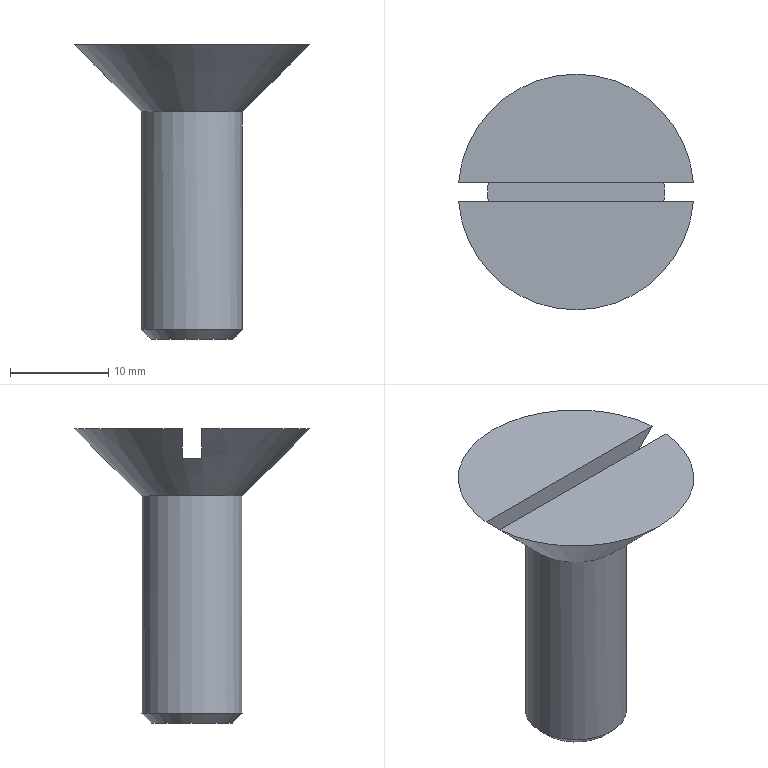Component | NX | COUNTER_SUNK_SCREW | 1 solid | 9 faces | box 23.92 x 24 x 30 mm | volume 3455 mm3 | plane 6 | cone 2 | cylinder 1 | commonest cylinder face diameters 10.3 x1
STEP:
#1=CARTESIAN_POINT('',(0.,0.,0.));
#2=DIRECTION('',(0.,0.,1.));
#3=DIRECTION('',(1.,0.,0.));
#4=AXIS2_PLACEMENT_3D('',#1,#2,#3);
#5=CARTESIAN_POINT('',(5.132,239.571,313.65));
#6=VERTEX_POINT('',#5);
#7=CARTESIAN_POINT('',(-5.15,240.,313.65));
#8=VERTEX_POINT('',#7);
#9=CARTESIAN_POINT('',(0.,240.,313.65));
#10=DIRECTION('',(0.,0.,-1.));
#11=DIRECTION('',(-1.,0.,0.));
#12=AXIS2_PLACEMENT_3D('',#9,#10,#11);
#13=CIRCLE('',#12,5.15);
#14=CARTESIAN_POINT('',(0.,240.,313.65));
#15=DIRECTION('',(0.,0.,1.));
#16=DIRECTION('',(1.,0.,0.));
#17=AXIS2_PLACEMENT_3D('',#14,#15,#16);
#18=CONICAL_SURFACE('',#17,5.15,0.7854);
#19=CARTESIAN_POINT('',(15.708,0.));
#20=DIRECTION('',(-1.,0.));
#21=VECTOR('',#20,1.);
#22=LINE('',#19,#21);
#23=(GEOMETRIC_REPRESENTATION_CONTEXT(2)PARAMETRIC_REPRESENTATION_CONTEXT()REPRESENTATION_CONTEXT('',''));
#24=DEFINITIONAL_REPRESENTATION('',(#22),#23);
#25=PCURVE('',#18,#24);
#26=CARTESIAN_POINT('',(0.,240.,290.5));
#27=DIRECTION('',(0.,0.,-1.));
#28=DIRECTION('',(-1.,0.,0.));
#29=AXIS2_PLACEMENT_3D('',#26,#27,#28);
#30=CYLINDRICAL_SURFACE('',#29,5.15);
#31=CARTESIAN_POINT('',(0.,-23.15));
#32=DIRECTION('',(1.,0.));
#33=VECTOR('',#32,1.);
#34=LINE('',#31,#33);
#35=(GEOMETRIC_REPRESENTATION_CONTEXT(2)PARAMETRIC_REPRESENTATION_CONTEXT()REPRESENTATION_CONTEXT('',''));
#36=DEFINITIONAL_REPRESENTATION('',(#34),#35);
#37=PCURVE('',#30,#36);
#38=SURFACE_CURVE('',#13,(#25,#37),.PCURVE_S1.);
#39=EDGE_CURVE('',#6,#8,#38,.T.);
#40=ORIENTED_EDGE('',*,*,#39,.F.);
#41=CARTESIAN_POINT('',(8.969,239.25,317.5));
#42=VERTEX_POINT('',#41);
#43=CARTESIAN_POINT('',(5.132,239.571,313.65));
#44=CARTESIAN_POINT('',(8.969,239.25,317.5));
#45=B_SPLINE_CURVE_WITH_KNOTS('',1,(#43,#44),.UNSPECIFIED.,.F.,.F.,(2,2),(0.,5.445),.PIECEWISE_BEZIER_KNOTS.);
#46=CARTESIAN_POINT('',(12.483,0.));
#47=DIRECTION('',(0.,1.));
#48=VECTOR('',#47,1.);
#49=LINE('',#46,#48);
#50=(GEOMETRIC_REPRESENTATION_CONTEXT(2)PARAMETRIC_REPRESENTATION_CONTEXT()REPRESENTATION_CONTEXT('',''));
#51=DEFINITIONAL_REPRESENTATION('',(#49),#50);
#52=PCURVE('',#18,#51);
#53=CARTESIAN_POINT('',(6.2,0.));
#54=DIRECTION('',(0.,1.));
#55=VECTOR('',#54,1.);
#56=LINE('',#53,#55);
#57=(GEOMETRIC_REPRESENTATION_CONTEXT(2)PARAMETRIC_REPRESENTATION_CONTEXT()REPRESENTATION_CONTEXT('',''));
#58=DEFINITIONAL_REPRESENTATION('',(#56),#57);
#59=PCURVE('',#18,#58);
#60=SEAM_CURVE('',#45,(#52,#59),.PCURVE_S1.);
#61=EDGE_CURVE('',#6,#42,#60,.T.);
#62=ORIENTED_EDGE('',*,*,#61,.T.);
#63=CARTESIAN_POINT('',(8.944,239.,317.5));
#64=VERTEX_POINT('',#63);
#65=CARTESIAN_POINT('',(0.,240.,317.5));
#66=DIRECTION('',(0.,0.,-1.));
#67=DIRECTION('',(1.,0.,0.));
#68=AXIS2_PLACEMENT_3D('',#65,#66,#67);
#69=CIRCLE('',#68,9.);
#70=CARTESIAN_POINT('',(12.566,3.85));
#71=DIRECTION('',(-1.,0.));
#72=VECTOR('',#71,1.);
#73=LINE('',#70,#72);
#74=(GEOMETRIC_REPRESENTATION_CONTEXT(2)PARAMETRIC_REPRESENTATION_CONTEXT()REPRESENTATION_CONTEXT('',''));
#75=DEFINITIONAL_REPRESENTATION('',(#73),#74);
#76=PCURVE('',#18,#75);
#77=CARTESIAN_POINT('',(213.,239.,317.5));
#78=DIRECTION('',(0.,0.,1.));
#79=DIRECTION('',(1.,0.,0.));
#80=AXIS2_PLACEMENT_3D('',#77,#78,#79);
#81=PLANE('',#80);
#82=CARTESIAN_POINT('',(-204.,1.));
#83=CARTESIAN_POINT('',(-204.,-14.588));
#84=CARTESIAN_POINT('',(-217.5,-6.794));
#85=CARTESIAN_POINT('',(-231.,1.));
#86=CARTESIAN_POINT('',(-217.5,8.794));
#87=CARTESIAN_POINT('',(-204.,16.588));
#88=CARTESIAN_POINT('',(-204.,1.));
#89=(BOUNDED_CURVE()B_SPLINE_CURVE(2,(#82,#83,#84,#85,#86,#87,#88),.UNSPECIFIED.,.T.,.F.)B_SPLINE_CURVE_WITH_KNOTS((1,2,2,2,2,1),(-2.094,0.,2.094,4.189,6.283,8.378),.UNSPECIFIED.)CURVE()GEOMETRIC_REPRESENTATION_ITEM()RATIONAL_B_SPLINE_CURVE((1.,0.5,1.,0.5,1.,0.5,1.))REPRESENTATION_ITEM(''));
#90=(GEOMETRIC_REPRESENTATION_CONTEXT(2)PARAMETRIC_REPRESENTATION_CONTEXT()REPRESENTATION_CONTEXT('',''));
#91=DEFINITIONAL_REPRESENTATION('',(#89),#90);
#92=PCURVE('',#81,#91);
#93=SURFACE_CURVE('',#69,(#76,#92),.PCURVE_S1.);
#94=EDGE_CURVE('',#42,#64,#93,.T.);
#95=ORIENTED_EDGE('',*,*,#94,.T.);
#96=CARTESIAN_POINT('',(11.958,239.,320.5));
#97=VERTEX_POINT('',#96);
#98=CARTESIAN_POINT('',(8.944,239.,317.5));
#99=CARTESIAN_POINT('',(9.95,239.,318.499));
#100=CARTESIAN_POINT('',(10.954,239.,319.499));
#101=CARTESIAN_POINT('',(11.958,239.,320.5));
#102=B_SPLINE_CURVE_WITH_KNOTS('',3,(#98,#99,#100,#101),.UNSPECIFIED.,.F.,.F.,(4,4),(0.,1.),.PIECEWISE_BEZIER_KNOTS.);
#103=CARTESIAN_POINT('',(12.455,3.85));
#104=CARTESIAN_POINT('',(12.483,6.85));
#105=B_SPLINE_CURVE_WITH_KNOTS('',1,(#103,#104),.UNSPECIFIED.,.F.,.F.,(2,2),(0.,1.),.PIECEWISE_BEZIER_KNOTS.);
#106=(GEOMETRIC_REPRESENTATION_CONTEXT(2)PARAMETRIC_REPRESENTATION_CONTEXT()REPRESENTATION_CONTEXT('',''));
#107=DEFINITIONAL_REPRESENTATION('',(#105),#106);
#108=PCURVE('',#18,#107);
#109=CARTESIAN_POINT('',(213.,239.,324.5));
#110=DIRECTION('',(0.,1.,0.));
#111=DIRECTION('',(0.,-0.,1.));
#112=AXIS2_PLACEMENT_3D('',#109,#110,#111);
#113=PLANE('',#112);
#114=CARTESIAN_POINT('',(-7.,-204.056));
#115=CARTESIAN_POINT('',(-6.001,-203.05));
#116=CARTESIAN_POINT('',(-5.001,-202.046));
#117=CARTESIAN_POINT('',(-4.,-201.042));
#118=B_SPLINE_CURVE_WITH_KNOTS('',3,(#114,#115,#116,#117),.UNSPECIFIED.,.F.,.F.,(4,4),(0.,1.),.PIECEWISE_BEZIER_KNOTS.);
#119=(GEOMETRIC_REPRESENTATION_CONTEXT(2)PARAMETRIC_REPRESENTATION_CONTEXT()REPRESENTATION_CONTEXT('',''));
#120=DEFINITIONAL_REPRESENTATION('',(#118),#119);
#121=PCURVE('',#113,#120);
#122=SURFACE_CURVE('',#102,(#108,#121),.PCURVE_S1.);
#123=EDGE_CURVE('',#64,#97,#122,.T.);
#124=ORIENTED_EDGE('',*,*,#123,.T.);
#125=CARTESIAN_POINT('',(-11.958,239.,320.5));
#126=VERTEX_POINT('',#125);
#127=CARTESIAN_POINT('',(0.,240.,320.5));
#128=DIRECTION('',(0.,0.,-1.));
#129=DIRECTION('',(-1.,0.,0.));
#130=AXIS2_PLACEMENT_3D('',#127,#128,#129);
#131=CIRCLE('',#130,12.);
#132=CARTESIAN_POINT('',(15.708,6.85));
#133=DIRECTION('',(-1.,0.));
#134=VECTOR('',#133,1.);
#135=LINE('',#132,#134);
#136=(GEOMETRIC_REPRESENTATION_CONTEXT(2)PARAMETRIC_REPRESENTATION_CONTEXT()REPRESENTATION_CONTEXT('',''));
#137=DEFINITIONAL_REPRESENTATION('',(#135),#136);
#138=PCURVE('',#18,#137);
#139=CARTESIAN_POINT('',(12.,240.,320.5));
#140=DIRECTION('',(0.,0.,1.));
#141=DIRECTION('',(1.,0.,0.));
#142=AXIS2_PLACEMENT_3D('',#139,#140,#141);
#143=PLANE('',#142);
#144=CARTESIAN_POINT('',(-24.,0.));
#145=CARTESIAN_POINT('',(-24.,20.785));
#146=CARTESIAN_POINT('',(-6.,10.392));
#147=CARTESIAN_POINT('',(12.,0.));
#148=CARTESIAN_POINT('',(-6.,-10.392));
#149=CARTESIAN_POINT('',(-24.,-20.785));
#150=CARTESIAN_POINT('',(-24.,0.));
#151=(BOUNDED_CURVE()B_SPLINE_CURVE(2,(#144,#145,#146,#147,#148,#149,#150),.UNSPECIFIED.,.T.,.F.)B_SPLINE_CURVE_WITH_KNOTS((1,2,2,2,2,1),(-2.094,0.,2.094,4.189,6.283,8.378),.UNSPECIFIED.)CURVE()GEOMETRIC_REPRESENTATION_ITEM()RATIONAL_B_SPLINE_CURVE((1.,0.5,1.,0.5,1.,0.5,1.))REPRESENTATION_ITEM(''));
#152=(GEOMETRIC_REPRESENTATION_CONTEXT(2)PARAMETRIC_REPRESENTATION_CONTEXT()REPRESENTATION_CONTEXT('',''));
#153=DEFINITIONAL_REPRESENTATION('',(#151),#152);
#154=PCURVE('',#143,#153);
#155=SURFACE_CURVE('',#131,(#138,#154),.PCURVE_S1.);
#156=EDGE_CURVE('',#97,#126,#155,.T.);
#157=ORIENTED_EDGE('',*,*,#156,.T.);
#158=CARTESIAN_POINT('',(-8.944,239.,317.5));
#159=VERTEX_POINT('',#158);
#160=CARTESIAN_POINT('',(-11.958,239.,320.5));
#161=CARTESIAN_POINT('',(-10.954,239.,319.499));
#162=CARTESIAN_POINT('',(-9.95,239.,318.499));
#163=CARTESIAN_POINT('',(-8.944,239.,317.5));
#164=B_SPLINE_CURVE_WITH_KNOTS('',3,(#160,#161,#162,#163),.UNSPECIFIED.,.F.,.F.,(4,4),(0.,1.),.PIECEWISE_BEZIER_KNOTS.);
#165=CARTESIAN_POINT('',(9.508,6.85));
#166=CARTESIAN_POINT('',(9.536,3.85));
#167=B_SPLINE_CURVE_WITH_KNOTS('',1,(#165,#166),.UNSPECIFIED.,.F.,.F.,(2,2),(0.,1.),.PIECEWISE_BEZIER_KNOTS.);
#168=(GEOMETRIC_REPRESENTATION_CONTEXT(2)PARAMETRIC_REPRESENTATION_CONTEXT()REPRESENTATION_CONTEXT('',''));
#169=DEFINITIONAL_REPRESENTATION('',(#167),#168);
#170=PCURVE('',#18,#169);
#171=CARTESIAN_POINT('',(-4.,-224.958));
#172=CARTESIAN_POINT('',(-5.001,-223.954));
#173=CARTESIAN_POINT('',(-6.001,-222.95));
#174=CARTESIAN_POINT('',(-7.,-221.944));
#175=B_SPLINE_CURVE_WITH_KNOTS('',3,(#171,#172,#173,#174),.UNSPECIFIED.,.F.,.F.,(4,4),(0.,1.),.PIECEWISE_BEZIER_KNOTS.);
#176=(GEOMETRIC_REPRESENTATION_CONTEXT(2)PARAMETRIC_REPRESENTATION_CONTEXT()REPRESENTATION_CONTEXT('',''));
#177=DEFINITIONAL_REPRESENTATION('',(#175),#176);
#178=PCURVE('',#113,#177);
#179=SURFACE_CURVE('',#164,(#170,#178),.PCURVE_S1.);
#180=EDGE_CURVE('',#126,#159,#179,.T.);
#181=ORIENTED_EDGE('',*,*,#180,.T.);
#182=CARTESIAN_POINT('',(-8.944,241.,317.5));
#183=VERTEX_POINT('',#182);
#184=CARTESIAN_POINT('',(0.,240.,317.5));
#185=DIRECTION('',(0.,0.,-1.));
#186=DIRECTION('',(1.,0.,0.));
#187=AXIS2_PLACEMENT_3D('',#184,#185,#186);
#188=CIRCLE('',#187,9.);
#189=CARTESIAN_POINT('',(12.566,3.85));
#190=DIRECTION('',(-1.,0.));
#191=VECTOR('',#190,1.);
#192=LINE('',#189,#191);
#193=(GEOMETRIC_REPRESENTATION_CONTEXT(2)PARAMETRIC_REPRESENTATION_CONTEXT()REPRESENTATION_CONTEXT('',''));
#194=DEFINITIONAL_REPRESENTATION('',(#192),#193);
#195=PCURVE('',#18,#194);
#196=CARTESIAN_POINT('',(-204.,1.));
#197=CARTESIAN_POINT('',(-204.,-14.588));
#198=CARTESIAN_POINT('',(-217.5,-6.794));
#199=CARTESIAN_POINT('',(-231.,1.));
#200=CARTESIAN_POINT('',(-217.5,8.794));
#201=CARTESIAN_POINT('',(-204.,16.588));
#202=CARTESIAN_POINT('',(-204.,1.));
#203=(BOUNDED_CURVE()B_SPLINE_CURVE(2,(#196,#197,#198,#199,#200,#201,#202),.UNSPECIFIED.,.T.,.F.)B_SPLINE_CURVE_WITH_KNOTS((1,2,2,2,2,1),(-2.094,0.,2.094,4.189,6.283,8.378),.UNSPECIFIED.)CURVE()GEOMETRIC_REPRESENTATION_ITEM()RATIONAL_B_SPLINE_CURVE((1.,0.5,1.,0.5,1.,0.5,1.))REPRESENTATION_ITEM(''));
#204=(GEOMETRIC_REPRESENTATION_CONTEXT(2)PARAMETRIC_REPRESENTATION_CONTEXT()REPRESENTATION_CONTEXT('',''));
#205=DEFINITIONAL_REPRESENTATION('',(#203),#204);
#206=PCURVE('',#81,#205);
#207=SURFACE_CURVE('',#188,(#195,#206),.PCURVE_S1.);
#208=EDGE_CURVE('',#159,#183,#207,.T.);
#209=ORIENTED_EDGE('',*,*,#208,.T.);
#210=CARTESIAN_POINT('',(-11.958,241.,320.5));
#211=VERTEX_POINT('',#210);
#212=CARTESIAN_POINT('',(-8.944,241.,317.5));
#213=CARTESIAN_POINT('',(-9.95,241.,318.499));
#214=CARTESIAN_POINT('',(-10.954,241.,319.499));
#215=CARTESIAN_POINT('',(-11.958,241.,320.5));
#216=B_SPLINE_CURVE_WITH_KNOTS('',3,(#212,#213,#214,#215),.UNSPECIFIED.,.F.,.F.,(4,4),(0.,1.),.PIECEWISE_BEZIER_KNOTS.);
#217=CARTESIAN_POINT('',(9.313,3.85));
#218=CARTESIAN_POINT('',(9.341,6.85));
#219=B_SPLINE_CURVE_WITH_KNOTS('',1,(#217,#218),.UNSPECIFIED.,.F.,.F.,(2,2),(0.,1.),.PIECEWISE_BEZIER_KNOTS.);
#220=(GEOMETRIC_REPRESENTATION_CONTEXT(2)PARAMETRIC_REPRESENTATION_CONTEXT()REPRESENTATION_CONTEXT('',''));
#221=DEFINITIONAL_REPRESENTATION('',(#219),#220);
#222=PCURVE('',#18,#221);
#223=CARTESIAN_POINT('',(213.,241.,317.5));
#224=DIRECTION('',(0.,-1.,-0.));
#225=DIRECTION('',(0.,0.,-1.));
#226=AXIS2_PLACEMENT_3D('',#223,#224,#225);
#227=PLANE('',#226);
#228=CARTESIAN_POINT('',(0.,-221.944));
#229=CARTESIAN_POINT('',(-0.9992,-222.95));
#230=CARTESIAN_POINT('',(-1.999,-223.954));
#231=CARTESIAN_POINT('',(-3.,-224.958));
#232=B_SPLINE_CURVE_WITH_KNOTS('',3,(#228,#229,#230,#231),.UNSPECIFIED.,.F.,.F.,(4,4),(0.,1.),.PIECEWISE_BEZIER_KNOTS.);
#233=(GEOMETRIC_REPRESENTATION_CONTEXT(2)PARAMETRIC_REPRESENTATION_CONTEXT()REPRESENTATION_CONTEXT('',''));
#234=DEFINITIONAL_REPRESENTATION('',(#232),#233);
#235=PCURVE('',#227,#234);
#236=SURFACE_CURVE('',#216,(#222,#235),.PCURVE_S1.);
#237=EDGE_CURVE('',#183,#211,#236,.T.);
#238=ORIENTED_EDGE('',*,*,#237,.T.);
#239=CARTESIAN_POINT('',(11.958,241.,320.5));
#240=VERTEX_POINT('',#239);
#241=CARTESIAN_POINT('',(0.,240.,320.5));
#242=DIRECTION('',(0.,0.,-1.));
#243=DIRECTION('',(-1.,0.,0.));
#244=AXIS2_PLACEMENT_3D('',#241,#242,#243);
#245=CIRCLE('',#244,12.);
#246=CARTESIAN_POINT('',(9.425,6.85));
#247=DIRECTION('',(-1.,0.));
#248=VECTOR('',#247,1.);
#249=LINE('',#246,#248);
#250=(GEOMETRIC_REPRESENTATION_CONTEXT(2)PARAMETRIC_REPRESENTATION_CONTEXT()REPRESENTATION_CONTEXT('',''));
#251=DEFINITIONAL_REPRESENTATION('',(#249),#250);
#252=PCURVE('',#18,#251);
#253=CARTESIAN_POINT('',(12.,240.,320.5));
#254=DIRECTION('',(0.,0.,1.));
#255=DIRECTION('',(1.,0.,0.));
#256=AXIS2_PLACEMENT_3D('',#253,#254,#255);
#257=PLANE('',#256);
#258=CARTESIAN_POINT('',(-24.,0.));
#259=CARTESIAN_POINT('',(-24.,20.785));
#260=CARTESIAN_POINT('',(-6.,10.392));
#261=CARTESIAN_POINT('',(12.,0.));
#262=CARTESIAN_POINT('',(-6.,-10.392));
#263=CARTESIAN_POINT('',(-24.,-20.785));
#264=CARTESIAN_POINT('',(-24.,0.));
#265=(BOUNDED_CURVE()B_SPLINE_CURVE(2,(#258,#259,#260,#261,#262,#263,#264),.UNSPECIFIED.,.T.,.F.)B_SPLINE_CURVE_WITH_KNOTS((1,2,2,2,2,1),(-2.094,0.,2.094,4.189,6.283,8.378),.UNSPECIFIED.)CURVE()GEOMETRIC_REPRESENTATION_ITEM()RATIONAL_B_SPLINE_CURVE((1.,0.5,1.,0.5,1.,0.5,1.))REPRESENTATION_ITEM(''));
#266=(GEOMETRIC_REPRESENTATION_CONTEXT(2)PARAMETRIC_REPRESENTATION_CONTEXT()REPRESENTATION_CONTEXT('',''));
#267=DEFINITIONAL_REPRESENTATION('',(#265),#266);
#268=PCURVE('',#257,#267);
#269=SURFACE_CURVE('',#245,(#252,#268),.PCURVE_S1.);
#270=EDGE_CURVE('',#211,#240,#269,.T.);
#271=ORIENTED_EDGE('',*,*,#270,.T.);
#272=CARTESIAN_POINT('',(8.944,241.,317.5));
#273=VERTEX_POINT('',#272);
#274=CARTESIAN_POINT('',(11.958,241.,320.5));
#275=CARTESIAN_POINT('',(10.954,241.,319.499));
#276=CARTESIAN_POINT('',(9.95,241.,318.499));
#277=CARTESIAN_POINT('',(8.944,241.,317.5));
#278=B_SPLINE_CURVE_WITH_KNOTS('',3,(#274,#275,#276,#277),.UNSPECIFIED.,.F.,.F.,(4,4),(0.,1.),.PIECEWISE_BEZIER_KNOTS.);
#279=CARTESIAN_POINT('',(6.367,6.85));
#280=CARTESIAN_POINT('',(6.395,3.85));
#281=B_SPLINE_CURVE_WITH_KNOTS('',1,(#279,#280),.UNSPECIFIED.,.F.,.F.,(2,2),(0.,1.),.PIECEWISE_BEZIER_KNOTS.);
#282=(GEOMETRIC_REPRESENTATION_CONTEXT(2)PARAMETRIC_REPRESENTATION_CONTEXT()REPRESENTATION_CONTEXT('',''));
#283=DEFINITIONAL_REPRESENTATION('',(#281),#282);
#284=PCURVE('',#18,#283);
#285=CARTESIAN_POINT('',(-3.,-201.042));
#286=CARTESIAN_POINT('',(-1.999,-202.046));
#287=CARTESIAN_POINT('',(-0.9992,-203.05));
#288=CARTESIAN_POINT('',(0.,-204.056));
#289=B_SPLINE_CURVE_WITH_KNOTS('',3,(#285,#286,#287,#288),.UNSPECIFIED.,.F.,.F.,(4,4),(0.,1.),.PIECEWISE_BEZIER_KNOTS.);
#290=(GEOMETRIC_REPRESENTATION_CONTEXT(2)PARAMETRIC_REPRESENTATION_CONTEXT()REPRESENTATION_CONTEXT('',''));
#291=DEFINITIONAL_REPRESENTATION('',(#289),#290);
#292=PCURVE('',#227,#291);
#293=SURFACE_CURVE('',#278,(#284,#292),.PCURVE_S1.);
#294=EDGE_CURVE('',#240,#273,#293,.T.);
#295=ORIENTED_EDGE('',*,*,#294,.T.);
#296=CARTESIAN_POINT('',(0.,240.,317.5));
#297=DIRECTION('',(0.,0.,-1.));
#298=DIRECTION('',(1.,0.,0.));
#299=AXIS2_PLACEMENT_3D('',#296,#297,#298);
#300=CIRCLE('',#299,9.);
#301=CARTESIAN_POINT('',(12.566,3.85));
#302=DIRECTION('',(-1.,0.));
#303=VECTOR('',#302,1.);
#304=LINE('',#301,#303);
#305=(GEOMETRIC_REPRESENTATION_CONTEXT(2)PARAMETRIC_REPRESENTATION_CONTEXT()REPRESENTATION_CONTEXT('',''));
#306=DEFINITIONAL_REPRESENTATION('',(#304),#305);
#307=PCURVE('',#18,#306);
#308=CARTESIAN_POINT('',(-204.,1.));
#309=CARTESIAN_POINT('',(-204.,-14.588));
#310=CARTESIAN_POINT('',(-217.5,-6.794));
#311=CARTESIAN_POINT('',(-231.,1.));
#312=CARTESIAN_POINT('',(-217.5,8.794));
#313=CARTESIAN_POINT('',(-204.,16.588));
#314=CARTESIAN_POINT('',(-204.,1.));
#315=(BOUNDED_CURVE()B_SPLINE_CURVE(2,(#308,#309,#310,#311,#312,#313,#314),.UNSPECIFIED.,.T.,.F.)B_SPLINE_CURVE_WITH_KNOTS((1,2,2,2,2,1),(-2.094,0.,2.094,4.189,6.283,8.378),.UNSPECIFIED.)CURVE()GEOMETRIC_REPRESENTATION_ITEM()RATIONAL_B_SPLINE_CURVE((1.,0.5,1.,0.5,1.,0.5,1.))REPRESENTATION_ITEM(''));
#316=(GEOMETRIC_REPRESENTATION_CONTEXT(2)PARAMETRIC_REPRESENTATION_CONTEXT()REPRESENTATION_CONTEXT('',''));
#317=DEFINITIONAL_REPRESENTATION('',(#315),#316);
#318=PCURVE('',#81,#317);
#319=SURFACE_CURVE('',#300,(#307,#318),.PCURVE_S1.);
#320=EDGE_CURVE('',#273,#42,#319,.T.);
#321=ORIENTED_EDGE('',*,*,#320,.T.);
#322=ORIENTED_EDGE('',*,*,#61,.F.);
#323=CARTESIAN_POINT('',(0.,240.,313.65));
#324=DIRECTION('',(0.,0.,-1.));
#325=DIRECTION('',(-1.,0.,0.));
#326=AXIS2_PLACEMENT_3D('',#323,#324,#325);
#327=CIRCLE('',#326,5.15);
#328=CARTESIAN_POINT('',(9.425,0.));
#329=DIRECTION('',(-1.,0.));
#330=VECTOR('',#329,1.);
#331=LINE('',#328,#330);
#332=(GEOMETRIC_REPRESENTATION_CONTEXT(2)PARAMETRIC_REPRESENTATION_CONTEXT()REPRESENTATION_CONTEXT('',''));
#333=DEFINITIONAL_REPRESENTATION('',(#331),#332);
#334=PCURVE('',#18,#333);
#335=CARTESIAN_POINT('',(0.,-23.15));
#336=DIRECTION('',(1.,0.));
#337=VECTOR('',#336,1.);
#338=LINE('',#335,#337);
#339=(GEOMETRIC_REPRESENTATION_CONTEXT(2)PARAMETRIC_REPRESENTATION_CONTEXT()REPRESENTATION_CONTEXT('',''));
#340=DEFINITIONAL_REPRESENTATION('',(#338),#339);
#341=PCURVE('',#30,#340);
#342=SURFACE_CURVE('',#327,(#334,#341),.PCURVE_S1.);
#343=EDGE_CURVE('',#8,#6,#342,.T.);
#344=ORIENTED_EDGE('',*,*,#343,.F.);
#345=EDGE_LOOP('',(#40,#62,#95,#124,#157,#181,#209,#238,#271,#295,#321,#322,#344));
#346=FACE_BOUND('',#345,.T.);
#347=ADVANCED_FACE('',(#346),#18,.T.);
#348=ORIENTED_EDGE('',*,*,#156,.F.);
#349=CARTESIAN_POINT('',(12.,239.,320.5));
#350=DIRECTION('',(-1.,0.,0.));
#351=VECTOR('',#350,1.);
#352=LINE('',#349,#351);
#353=CARTESIAN_POINT('',(0.,-1.));
#354=DIRECTION('',(-1.,0.));
#355=VECTOR('',#354,1.);
#356=LINE('',#353,#355);
#357=(GEOMETRIC_REPRESENTATION_CONTEXT(2)PARAMETRIC_REPRESENTATION_CONTEXT()REPRESENTATION_CONTEXT('',''));
#358=DEFINITIONAL_REPRESENTATION('',(#356),#357);
#359=PCURVE('',#143,#358);
#360=CARTESIAN_POINT('',(-4.,-201.));
#361=DIRECTION('',(0.,-1.));
#362=VECTOR('',#361,1.);
#363=LINE('',#360,#362);
#364=(GEOMETRIC_REPRESENTATION_CONTEXT(2)PARAMETRIC_REPRESENTATION_CONTEXT()REPRESENTATION_CONTEXT('',''));
#365=DEFINITIONAL_REPRESENTATION('',(#363),#364);
#366=PCURVE('',#113,#365);
#367=SURFACE_CURVE('',#352,(#359,#366),.PCURVE_S1.);
#368=EDGE_CURVE('',#97,#126,#367,.T.);
#369=ORIENTED_EDGE('',*,*,#368,.T.);
#370=EDGE_LOOP('',(#348,#369));
#371=FACE_BOUND('',#370,.T.);
#372=ADVANCED_FACE('',(#371),#143,.T.);
#373=ORIENTED_EDGE('',*,*,#270,.F.);
#374=CARTESIAN_POINT('',(12.,241.,320.5));
#375=DIRECTION('',(1.,0.,0.));
#376=VECTOR('',#375,1.);
#377=LINE('',#374,#376);
#378=CARTESIAN_POINT('',(0.,1.));
#379=DIRECTION('',(1.,0.));
#380=VECTOR('',#379,1.);
#381=LINE('',#378,#380);
#382=(GEOMETRIC_REPRESENTATION_CONTEXT(2)PARAMETRIC_REPRESENTATION_CONTEXT()REPRESENTATION_CONTEXT('',''));
#383=DEFINITIONAL_REPRESENTATION('',(#381),#382);
#384=PCURVE('',#257,#383);
#385=CARTESIAN_POINT('',(-3.,-201.));
#386=DIRECTION('',(0.,1.));
#387=VECTOR('',#386,1.);
#388=LINE('',#385,#387);
#389=(GEOMETRIC_REPRESENTATION_CONTEXT(2)PARAMETRIC_REPRESENTATION_CONTEXT()REPRESENTATION_CONTEXT('',''));
#390=DEFINITIONAL_REPRESENTATION('',(#388),#389);
#391=PCURVE('',#227,#390);
#392=SURFACE_CURVE('',#377,(#384,#391),.PCURVE_S1.);
#393=EDGE_CURVE('',#211,#240,#392,.T.);
#394=ORIENTED_EDGE('',*,*,#393,.T.);
#395=EDGE_LOOP('',(#373,#394));
#396=FACE_BOUND('',#395,.T.);
#397=ADVANCED_FACE('',(#396),#257,.T.);
#398=CARTESIAN_POINT('',(-4.15,240.,290.5));
#399=VERTEX_POINT('',#398);
#400=CARTESIAN_POINT('',(0.,240.,290.5));
#401=DIRECTION('',(0.,0.,-1.));
#402=DIRECTION('',(-1.,0.,0.));
#403=AXIS2_PLACEMENT_3D('',#400,#401,#402);
#404=CIRCLE('',#403,4.15);
#405=CARTESIAN_POINT('',(0.,240.,290.5));
#406=DIRECTION('',(0.,0.,-1.));
#407=DIRECTION('',(-1.,0.,0.));
#408=AXIS2_PLACEMENT_3D('',#405,#406,#407);
#409=PLANE('',#408);
#410=CARTESIAN_POINT('',(0.,0.));
#411=DIRECTION('',(1.,0.));
#412=AXIS2_PLACEMENT_2D('',#410,#411);
#413=CIRCLE('',#412,4.15);
#414=(GEOMETRIC_REPRESENTATION_CONTEXT(2)PARAMETRIC_REPRESENTATION_CONTEXT()REPRESENTATION_CONTEXT('',''));
#415=DEFINITIONAL_REPRESENTATION('',(#413),#414);
#416=PCURVE('',#409,#415);
#417=CARTESIAN_POINT('',(0.,240.,290.5));
#418=DIRECTION('',(0.,0.,1.));
#419=DIRECTION('',(1.,0.,0.));
#420=AXIS2_PLACEMENT_3D('',#417,#418,#419);
#421=CONICAL_SURFACE('',#420,4.15,0.7854);
#422=CARTESIAN_POINT('',(9.425,0.));
#423=DIRECTION('',(-1.,0.));
#424=VECTOR('',#423,1.);
#425=LINE('',#422,#424);
#426=(GEOMETRIC_REPRESENTATION_CONTEXT(2)PARAMETRIC_REPRESENTATION_CONTEXT()REPRESENTATION_CONTEXT('',''));
#427=DEFINITIONAL_REPRESENTATION('',(#425),#426);
#428=PCURVE('',#421,#427);
#429=SURFACE_CURVE('',#404,(#416,#428),.PCURVE_S1.);
#430=EDGE_CURVE('',#399,#399,#429,.T.);
#431=ORIENTED_EDGE('',*,*,#430,.T.);
#432=EDGE_LOOP('',(#431));
#433=FACE_BOUND('',#432,.T.);
#434=ADVANCED_FACE('',(#433),#409,.T.);
#435=CARTESIAN_POINT('',(-5.15,240.,291.5));
#436=VERTEX_POINT('',#435);
#437=CARTESIAN_POINT('',(0.,240.,291.5));
#438=DIRECTION('',(0.,0.,1.));
#439=DIRECTION('',(-1.,0.,0.));
#440=AXIS2_PLACEMENT_3D('',#437,#438,#439);
#441=CIRCLE('',#440,5.15);
#442=CARTESIAN_POINT('',(6.283,-1.));
#443=DIRECTION('',(-1.,0.));
#444=VECTOR('',#443,1.);
#445=LINE('',#442,#444);
#446=(GEOMETRIC_REPRESENTATION_CONTEXT(2)PARAMETRIC_REPRESENTATION_CONTEXT()REPRESENTATION_CONTEXT('',''));
#447=DEFINITIONAL_REPRESENTATION('',(#445),#446);
#448=PCURVE('',#30,#447);
#449=CARTESIAN_POINT('',(3.142,1.));
#450=DIRECTION('',(1.,0.));
#451=VECTOR('',#450,1.);
#452=LINE('',#449,#451);
#453=(GEOMETRIC_REPRESENTATION_CONTEXT(2)PARAMETRIC_REPRESENTATION_CONTEXT()REPRESENTATION_CONTEXT('',''));
#454=DEFINITIONAL_REPRESENTATION('',(#452),#453);
#455=PCURVE('',#421,#454);
#456=SURFACE_CURVE('',#441,(#448,#455),.PCURVE_S1.);
#457=EDGE_CURVE('',#436,#436,#456,.T.);
#458=ORIENTED_EDGE('',*,*,#457,.T.);
#459=CARTESIAN_POINT('',(-5.15,240.,313.65));
#460=CARTESIAN_POINT('',(-5.15,240.,291.5));
#461=B_SPLINE_CURVE_WITH_KNOTS('',1,(#459,#460),.UNSPECIFIED.,.F.,.F.,(2,2),(-23.15,-1.),.PIECEWISE_BEZIER_KNOTS.);
#462=CARTESIAN_POINT('',(0.,0.));
#463=DIRECTION('',(0.,1.));
#464=VECTOR('',#463,1.);
#465=LINE('',#462,#464);
#466=(GEOMETRIC_REPRESENTATION_CONTEXT(2)PARAMETRIC_REPRESENTATION_CONTEXT()REPRESENTATION_CONTEXT('',''));
#467=DEFINITIONAL_REPRESENTATION('',(#465),#466);
#468=PCURVE('',#30,#467);
#469=CARTESIAN_POINT('',(6.283,0.));
#470=DIRECTION('',(0.,1.));
#471=VECTOR('',#470,1.);
#472=LINE('',#469,#471);
#473=(GEOMETRIC_REPRESENTATION_CONTEXT(2)PARAMETRIC_REPRESENTATION_CONTEXT()REPRESENTATION_CONTEXT('',''));
#474=DEFINITIONAL_REPRESENTATION('',(#472),#473);
#475=PCURVE('',#30,#474);
#476=SEAM_CURVE('',#461,(#468,#475),.PCURVE_S1.);
#477=EDGE_CURVE('',#8,#436,#476,.T.);
#478=ORIENTED_EDGE('',*,*,#477,.F.);
#479=ORIENTED_EDGE('',*,*,#343,.T.);
#480=ORIENTED_EDGE('',*,*,#39,.T.);
#481=ORIENTED_EDGE('',*,*,#477,.T.);
#482=EDGE_LOOP('',(#458,#478,#479,#480,#481));
#483=FACE_BOUND('',#482,.T.);
#484=ADVANCED_FACE('',(#483),#30,.T.);
#485=ORIENTED_EDGE('',*,*,#368,.F.);
#486=ORIENTED_EDGE('',*,*,#123,.F.);
#487=CARTESIAN_POINT('',(213.,239.,317.5));
#488=DIRECTION('',(1.,0.,0.));
#489=VECTOR('',#488,1.);
#490=LINE('',#487,#489);
#491=CARTESIAN_POINT('',(-7.,0.));
#492=DIRECTION('',(0.,1.));
#493=VECTOR('',#492,1.);
#494=LINE('',#491,#493);
#495=(GEOMETRIC_REPRESENTATION_CONTEXT(2)PARAMETRIC_REPRESENTATION_CONTEXT()REPRESENTATION_CONTEXT('',''));
#496=DEFINITIONAL_REPRESENTATION('',(#494),#495);
#497=PCURVE('',#113,#496);
#498=CARTESIAN_POINT('',(0.,0.));
#499=DIRECTION('',(1.,0.));
#500=VECTOR('',#499,1.);
#501=LINE('',#498,#500);
#502=(GEOMETRIC_REPRESENTATION_CONTEXT(2)PARAMETRIC_REPRESENTATION_CONTEXT()REPRESENTATION_CONTEXT('',''));
#503=DEFINITIONAL_REPRESENTATION('',(#501),#502);
#504=PCURVE('',#81,#503);
#505=SURFACE_CURVE('',#490,(#497,#504),.PCURVE_S1.);
#506=EDGE_CURVE('',#159,#64,#505,.T.);
#507=ORIENTED_EDGE('',*,*,#506,.F.);
#508=ORIENTED_EDGE('',*,*,#180,.F.);
#509=EDGE_LOOP('',(#485,#486,#507,#508));
#510=FACE_BOUND('',#509,.T.);
#511=ADVANCED_FACE('',(#510),#113,.T.);
#512=ORIENTED_EDGE('',*,*,#506,.T.);
#513=ORIENTED_EDGE('',*,*,#94,.F.);
#514=ORIENTED_EDGE('',*,*,#320,.F.);
#515=CARTESIAN_POINT('',(213.,241.,317.5));
#516=DIRECTION('',(1.,0.,0.));
#517=VECTOR('',#516,1.);
#518=LINE('',#515,#517);
#519=CARTESIAN_POINT('',(0.,2.));
#520=DIRECTION('',(1.,0.));
#521=VECTOR('',#520,1.);
#522=LINE('',#519,#521);
#523=(GEOMETRIC_REPRESENTATION_CONTEXT(2)PARAMETRIC_REPRESENTATION_CONTEXT()REPRESENTATION_CONTEXT('',''));
#524=DEFINITIONAL_REPRESENTATION('',(#522),#523);
#525=PCURVE('',#81,#524);
#526=CARTESIAN_POINT('',(0.,0.));
#527=DIRECTION('',(0.,1.));
#528=VECTOR('',#527,1.);
#529=LINE('',#526,#528);
#530=(GEOMETRIC_REPRESENTATION_CONTEXT(2)PARAMETRIC_REPRESENTATION_CONTEXT()REPRESENTATION_CONTEXT('',''));
#531=DEFINITIONAL_REPRESENTATION('',(#529),#530);
#532=PCURVE('',#227,#531);
#533=SURFACE_CURVE('',#518,(#525,#532),.PCURVE_S1.);
#534=EDGE_CURVE('',#183,#273,#533,.T.);
#535=ORIENTED_EDGE('',*,*,#534,.F.);
#536=ORIENTED_EDGE('',*,*,#208,.F.);
#537=EDGE_LOOP('',(#512,#513,#514,#535,#536));
#538=FACE_BOUND('',#537,.T.);
#539=ADVANCED_FACE('',(#538),#81,.T.);
#540=ORIENTED_EDGE('',*,*,#393,.F.);
#541=ORIENTED_EDGE('',*,*,#237,.F.);
#542=ORIENTED_EDGE('',*,*,#534,.T.);
#543=ORIENTED_EDGE('',*,*,#294,.F.);
#544=EDGE_LOOP('',(#540,#541,#542,#543));
#545=FACE_BOUND('',#544,.T.);
#546=ADVANCED_FACE('',(#545),#227,.T.);
#547=ORIENTED_EDGE('',*,*,#457,.F.);
#548=CARTESIAN_POINT('',(-4.15,240.,290.5));
#549=CARTESIAN_POINT('',(-5.15,240.,291.5));
#550=B_SPLINE_CURVE_WITH_KNOTS('',1,(#548,#549),.UNSPECIFIED.,.F.,.F.,(2,2),(0.,1.414),.PIECEWISE_BEZIER_KNOTS.);
#551=CARTESIAN_POINT('',(3.142,0.));
#552=DIRECTION('',(0.,1.));
#553=VECTOR('',#552,1.);
#554=LINE('',#551,#553);
#555=(GEOMETRIC_REPRESENTATION_CONTEXT(2)PARAMETRIC_REPRESENTATION_CONTEXT()REPRESENTATION_CONTEXT('',''));
#556=DEFINITIONAL_REPRESENTATION('',(#554),#555);
#557=PCURVE('',#421,#556);
#558=CARTESIAN_POINT('',(9.425,0.));
#559=DIRECTION('',(0.,1.));
#560=VECTOR('',#559,1.);
#561=LINE('',#558,#560);
#562=(GEOMETRIC_REPRESENTATION_CONTEXT(2)PARAMETRIC_REPRESENTATION_CONTEXT()REPRESENTATION_CONTEXT('',''));
#563=DEFINITIONAL_REPRESENTATION('',(#561),#562);
#564=PCURVE('',#421,#563);
#565=SEAM_CURVE('',#550,(#557,#564),.PCURVE_S1.);
#566=EDGE_CURVE('',#399,#436,#565,.T.);
#567=ORIENTED_EDGE('',*,*,#566,.F.);
#568=ORIENTED_EDGE('',*,*,#430,.F.);
#569=ORIENTED_EDGE('',*,*,#566,.T.);
#570=EDGE_LOOP('',(#547,#567,#568,#569));
#571=FACE_BOUND('',#570,.T.);
#572=ADVANCED_FACE('',(#571),#421,.T.);
#573=CLOSED_SHELL('',(#347,#372,#397,#434,#484,#511,#539,#546,#572));
#574=MANIFOLD_SOLID_BREP('',#573);
#575=(LENGTH_UNIT()NAMED_UNIT(*)SI_UNIT(.MILLI.,.METRE.));
#576=UNCERTAINTY_MEASURE_WITH_UNIT(LENGTH_MEASURE(0.01),#575,'','');
#577=(NAMED_UNIT(*)PLANE_ANGLE_UNIT()SI_UNIT($,.RADIAN.));
#578=(NAMED_UNIT(*)SI_UNIT($,.STERADIAN.)SOLID_ANGLE_UNIT());
#579=(GEOMETRIC_REPRESENTATION_CONTEXT(3)GLOBAL_UNCERTAINTY_ASSIGNED_CONTEXT((#576))GLOBAL_UNIT_ASSIGNED_CONTEXT((#575,#577,#578))REPRESENTATION_CONTEXT('',''));
#580=ADVANCED_BREP_SHAPE_REPRESENTATION('',(#4,#574),#579);